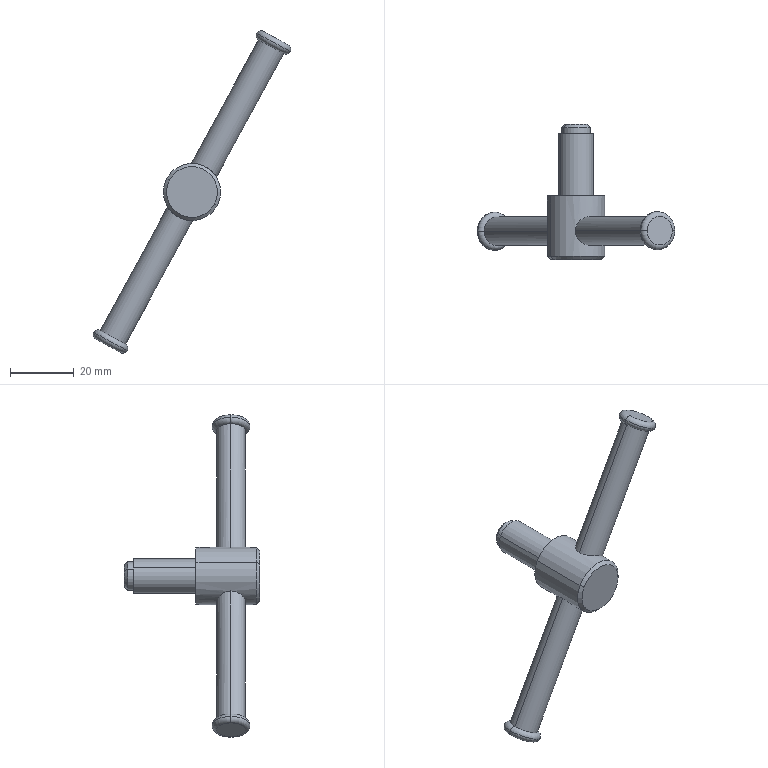Component | SolidWorks | 4-1 | 1 solid | 28 faces | box 62.09 x 42.5 x 101.27 mm | volume 13144 mm3 | cylinder 10 | torus 8 | plane 6 | cone 4 | commonest cylinder face diameters 9 x6 18 x2 10.8 x2
STEP:
#1=CARTESIAN_POINT('',(1.507,12.992,27.78));
#2=VERTEX_POINT('',#1);
#3=CARTESIAN_POINT('',(1.922,12.992,27.554));
#4=VERTEX_POINT('',#3);
#5=CARTESIAN_POINT('',(1.715,12.992,27.667));
#6=DIRECTION('',(-0.4783,-0.,-0.8782));
#7=DIRECTION('',(-0.8782,0.,0.4783));
#8=AXIS2_PLACEMENT_3D('',#5,#6,#7);
#9=CIRCLE('',#8,0.2362);
#10=EDGE_CURVE('',#2,#4,#9,.T.);
#11=ORIENTED_EDGE('',*,*,#10,.T.);
#12=CARTESIAN_POINT('',(1.842,12.992,27.53));
#13=VERTEX_POINT('',#12);
#14=CARTESIAN_POINT('',(1.87,12.992,27.582));
#15=DIRECTION('',(-0.,1.,-0.));
#16=DIRECTION('',(0.,0.,1.));
#17=AXIS2_PLACEMENT_3D('',#14,#15,#16);
#18=CIRCLE('',#17,0.05906);
#19=EDGE_CURVE('',#4,#13,#18,.T.);
#20=ORIENTED_EDGE('',*,*,#19,.T.);
#21=CARTESIAN_POINT('',(1.531,12.992,27.7));
#22=VERTEX_POINT('',#21);
#23=CARTESIAN_POINT('',(1.686,12.992,27.615));
#24=DIRECTION('',(0.4783,0.,0.8782));
#25=DIRECTION('',(0.8782,0.,-0.4783));
#26=AXIS2_PLACEMENT_3D('',#23,#24,#25);
#27=CIRCLE('',#26,0.1772);
#28=EDGE_CURVE('',#13,#22,#27,.T.);
#29=ORIENTED_EDGE('',*,*,#28,.T.);
#30=CARTESIAN_POINT('',(1.559,12.992,27.751));
#31=DIRECTION('',(0.,-1.,0.));
#32=DIRECTION('',(0.,0.,-1.));
#33=AXIS2_PLACEMENT_3D('',#30,#31,#32);
#34=CIRCLE('',#33,0.05906);
#35=EDGE_CURVE('',#2,#22,#34,.T.);
#36=ORIENTED_EDGE('',*,*,#35,.F.);
#37=EDGE_LOOP('',(#11,#20,#29,#36));
#38=FACE_OUTER_BOUND('',#37,.T.);
#39=CARTESIAN_POINT('',(1.715,12.992,27.667));
#40=DIRECTION('',(-0.4783,-0.,-0.8782));
#41=DIRECTION('',(-0.8782,-0.,0.4783));
#42=AXIS2_PLACEMENT_3D('',#39,#40,#41);
#43=TOROIDAL_SURFACE('',#42,0.1772,0.05906);
#44=ADVANCED_FACE('',(#38),#43,.T.);
#45=CARTESIAN_POINT('',(1.898,12.992,27.634));
#46=VERTEX_POINT('',#45);
#47=CARTESIAN_POINT('',(1.587,12.992,27.803));
#48=VERTEX_POINT('',#47);
#49=CARTESIAN_POINT('',(1.743,12.992,27.719));
#50=DIRECTION('',(0.4783,0.,0.8782));
#51=DIRECTION('',(-0.8782,0.,0.4783));
#52=AXIS2_PLACEMENT_3D('',#49,#50,#51);
#53=CIRCLE('',#52,0.1772);
#54=EDGE_CURVE('',#46,#48,#53,.T.);
#55=ORIENTED_EDGE('',*,*,#54,.F.);
#56=CARTESIAN_POINT('',(1.87,12.992,27.582));
#57=DIRECTION('',(-0.,1.,-0.));
#58=DIRECTION('',(0.,0.,1.));
#59=AXIS2_PLACEMENT_3D('',#56,#57,#58);
#60=CIRCLE('',#59,0.05906);
#61=EDGE_CURVE('',#46,#4,#60,.T.);
#62=ORIENTED_EDGE('',*,*,#61,.T.);
#63=ORIENTED_EDGE('',*,*,#10,.F.);
#64=CARTESIAN_POINT('',(1.559,12.992,27.751));
#65=DIRECTION('',(0.,-1.,0.));
#66=DIRECTION('',(0.,0.,-1.));
#67=AXIS2_PLACEMENT_3D('',#64,#65,#66);
#68=CIRCLE('',#67,0.05906);
#69=EDGE_CURVE('',#48,#2,#68,.T.);
#70=ORIENTED_EDGE('',*,*,#69,.F.);
#71=EDGE_LOOP('',(#55,#62,#63,#70));
#72=FACE_OUTER_BOUND('',#71,.T.);
#73=CARTESIAN_POINT('',(1.715,12.992,27.667));
#74=DIRECTION('',(-0.4783,-0.,-0.8782));
#75=DIRECTION('',(-0.8782,-0.,0.4783));
#76=AXIS2_PLACEMENT_3D('',#73,#74,#75);
#77=TOROIDAL_SURFACE('',#76,0.1772,0.05906);
#78=ADVANCED_FACE('',(#72),#77,.T.);
#79=CARTESIAN_POINT('',(1.009,12.992,26.002));
#80=VERTEX_POINT('',#79);
#81=CARTESIAN_POINT('',(0.6982,12.992,26.171));
#82=VERTEX_POINT('',#81);
#83=CARTESIAN_POINT('',(1.009,12.992,26.002));
#84=CARTESIAN_POINT('',(1.009,13.004,26.002));
#85=CARTESIAN_POINT('',(1.009,13.015,26.003));
#86=CARTESIAN_POINT('',(1.006,13.038,26.007));
#87=CARTESIAN_POINT('',(1.004,13.05,26.011));
#88=CARTESIAN_POINT('',(0.998,13.071,26.019));
#89=CARTESIAN_POINT('',(0.9946,13.081,26.024));
#90=CARTESIAN_POINT('',(0.9861,13.1,26.035));
#91=CARTESIAN_POINT('',(0.9812,13.109,26.042));
#92=CARTESIAN_POINT('',(0.97,13.125,26.055));
#93=CARTESIAN_POINT('',(0.9636,13.132,26.061));
#94=CARTESIAN_POINT('',(0.9495,13.145,26.075));
#95=CARTESIAN_POINT('',(0.9418,13.151,26.082));
#96=CARTESIAN_POINT('',(0.9251,13.16,26.096));
#97=CARTESIAN_POINT('',(0.916,13.163,26.103));
#98=CARTESIAN_POINT('',(0.8969,13.168,26.116));
#99=CARTESIAN_POINT('',(0.8869,13.169,26.122));
#100=CARTESIAN_POINT('',(0.8714,13.169,26.131));
#101=CARTESIAN_POINT('',(0.8661,13.169,26.134));
#102=CARTESIAN_POINT('',(0.8554,13.167,26.139));
#103=CARTESIAN_POINT('',(0.8501,13.167,26.141));
#104=CARTESIAN_POINT('',(0.8342,13.163,26.148));
#105=CARTESIAN_POINT('',(0.8235,13.16,26.152));
#106=CARTESIAN_POINT('',(0.8026,13.151,26.158));
#107=CARTESIAN_POINT('',(0.7925,13.145,26.161));
#108=CARTESIAN_POINT('',(0.7731,13.132,26.165));
#109=CARTESIAN_POINT('',(0.7638,13.125,26.167));
#110=CARTESIAN_POINT('',(0.7468,13.109,26.169));
#111=CARTESIAN_POINT('',(0.739,13.1,26.17));
#112=CARTESIAN_POINT('',(0.7249,13.081,26.171));
#113=CARTESIAN_POINT('',(0.7188,13.071,26.171));
#114=CARTESIAN_POINT('',(0.7088,13.05,26.171));
#115=CARTESIAN_POINT('',(0.7049,13.038,26.171));
#116=CARTESIAN_POINT('',(0.6995,13.015,26.171));
#117=CARTESIAN_POINT('',(0.6982,13.004,26.171));
#118=CARTESIAN_POINT('',(0.6982,12.992,26.171));
#119=B_SPLINE_CURVE_WITH_KNOTS('',3,(#83,#84,#85,#86,#87,#88,#89,#90,#91,#92,#93,#94,#95,#96,#97,#98,#99,#100,#101,#102,#103,#104,#105,#106,#107,#108,#109,#110,#111,#112,#113,#114,#115,#116,#117,#118),.UNSPECIFIED.,.F.,.F.,(4,2,2,2,2,2,2,2,2,2,2,2,2,2,2,2,2,4),(0.,0.0008945,0.001789,0.002684,0.003578,0.004473,0.005367,0.006262,0.007156,0.007604,0.008051,0.008945,0.00984,0.01073,0.01163,0.01252,0.01342,0.01431),.UNSPECIFIED.);
#120=EDGE_CURVE('',#80,#82,#119,.T.);
#121=ORIENTED_EDGE('',*,*,#120,.T.);
#122=CARTESIAN_POINT('',(0.5514,12.992,25.902));
#123=DIRECTION('',(0.4783,0.,0.8782));
#124=VECTOR('',#123,39.37);
#125=LINE('',#122,#124);
#126=EDGE_CURVE('',#82,#22,#125,.T.);
#127=ORIENTED_EDGE('',*,*,#126,.T.);
#128=ORIENTED_EDGE('',*,*,#28,.F.);
#129=CARTESIAN_POINT('',(0.8626,12.992,25.732));
#130=DIRECTION('',(0.4783,0.,0.8782));
#131=VECTOR('',#130,39.37);
#132=LINE('',#129,#131);
#133=EDGE_CURVE('',#80,#13,#132,.T.);
#134=ORIENTED_EDGE('',*,*,#133,.F.);
#135=EDGE_LOOP('',(#121,#127,#128,#134));
#136=FACE_OUTER_BOUND('',#135,.T.);
#137=CARTESIAN_POINT('',(0.707,12.992,25.817));
#138=DIRECTION('',(0.4783,0.,0.8782));
#139=DIRECTION('',(0.8782,0.,-0.4783));
#140=AXIS2_PLACEMENT_3D('',#137,#138,#139);
#141=CYLINDRICAL_SURFACE('',#140,0.1772);
#142=ADVANCED_FACE('',(#136),#141,.T.);
#143=CARTESIAN_POINT('',(-0.4844,12.992,24.));
#144=VERTEX_POINT('',#143);
#145=CARTESIAN_POINT('',(-0.1732,12.992,23.831));
#146=VERTEX_POINT('',#145);
#147=CARTESIAN_POINT('',(-0.3288,12.992,23.915));
#148=DIRECTION('',(-0.4783,-0.,-0.8782));
#149=DIRECTION('',(0.8782,0.,-0.4783));
#150=AXIS2_PLACEMENT_3D('',#147,#148,#149);
#151=CIRCLE('',#150,0.1772);
#152=EDGE_CURVE('',#144,#146,#151,.T.);
#153=ORIENTED_EDGE('',*,*,#152,.F.);
#154=CARTESIAN_POINT('',(-0.508,12.992,24.08));
#155=VERTEX_POINT('',#154);
#156=CARTESIAN_POINT('',(-0.4561,12.992,24.052));
#157=DIRECTION('',(0.,1.,-0.));
#158=DIRECTION('',(0.,0.,1.));
#159=AXIS2_PLACEMENT_3D('',#156,#157,#158);
#160=CIRCLE('',#159,0.05906);
#161=EDGE_CURVE('',#144,#155,#160,.T.);
#162=ORIENTED_EDGE('',*,*,#161,.T.);
#163=CARTESIAN_POINT('',(-0.09311,12.992,23.854));
#164=VERTEX_POINT('',#163);
#165=CARTESIAN_POINT('',(-0.3006,12.992,23.967));
#166=DIRECTION('',(-0.4783,-0.,-0.8782));
#167=DIRECTION('',(0.8782,0.,-0.4783));
#168=AXIS2_PLACEMENT_3D('',#165,#166,#167);
#169=CIRCLE('',#168,0.2362);
#170=EDGE_CURVE('',#155,#164,#169,.T.);
#171=ORIENTED_EDGE('',*,*,#170,.T.);
#172=CARTESIAN_POINT('',(-0.145,12.992,23.883));
#173=DIRECTION('',(0.,-1.,0.));
#174=DIRECTION('',(0.,0.,-1.));
#175=AXIS2_PLACEMENT_3D('',#172,#173,#174);
#176=CIRCLE('',#175,0.05906);
#177=EDGE_CURVE('',#146,#164,#176,.T.);
#178=ORIENTED_EDGE('',*,*,#177,.F.);
#179=EDGE_LOOP('',(#153,#162,#171,#178));
#180=FACE_OUTER_BOUND('',#179,.T.);
#181=CARTESIAN_POINT('',(-0.3006,12.992,23.967));
#182=DIRECTION('',(0.4783,0.,0.8782));
#183=DIRECTION('',(0.8782,0.,-0.4783));
#184=AXIS2_PLACEMENT_3D('',#181,#182,#183);
#185=TOROIDAL_SURFACE('',#184,0.1772,0.05906);
#186=ADVANCED_FACE('',(#180),#185,.T.);
#187=ORIENTED_EDGE('',*,*,#170,.F.);
#188=CARTESIAN_POINT('',(-0.4279,12.992,24.104));
#189=VERTEX_POINT('',#188);
#190=CARTESIAN_POINT('',(-0.4561,12.992,24.052));
#191=DIRECTION('',(0.,1.,-0.));
#192=DIRECTION('',(0.,0.,1.));
#193=AXIS2_PLACEMENT_3D('',#190,#191,#192);
#194=CIRCLE('',#193,0.05906);
#195=EDGE_CURVE('',#155,#189,#194,.T.);
#196=ORIENTED_EDGE('',*,*,#195,.T.);
#197=CARTESIAN_POINT('',(-0.1167,12.992,23.934));
#198=VERTEX_POINT('',#197);
#199=CARTESIAN_POINT('',(-0.2723,12.992,24.019));
#200=DIRECTION('',(0.4783,0.,0.8782));
#201=DIRECTION('',(0.8782,0.,-0.4783));
#202=AXIS2_PLACEMENT_3D('',#199,#200,#201);
#203=CIRCLE('',#202,0.1772);
#204=EDGE_CURVE('',#198,#189,#203,.T.);
#205=ORIENTED_EDGE('',*,*,#204,.F.);
#206=CARTESIAN_POINT('',(-0.145,12.992,23.883));
#207=DIRECTION('',(0.,-1.,0.));
#208=DIRECTION('',(0.,0.,-1.));
#209=AXIS2_PLACEMENT_3D('',#206,#207,#208);
#210=CIRCLE('',#209,0.05906);
#211=EDGE_CURVE('',#164,#198,#210,.T.);
#212=ORIENTED_EDGE('',*,*,#211,.F.);
#213=EDGE_LOOP('',(#187,#196,#205,#212));
#214=FACE_OUTER_BOUND('',#213,.T.);
#215=CARTESIAN_POINT('',(-0.3006,12.992,23.967));
#216=DIRECTION('',(0.4783,0.,0.8782));
#217=DIRECTION('',(0.8782,0.,-0.4783));
#218=AXIS2_PLACEMENT_3D('',#215,#216,#217);
#219=TOROIDAL_SURFACE('',#218,0.1772,0.05906);
#220=ADVANCED_FACE('',(#214),#219,.T.);
#221=CARTESIAN_POINT('',(0.586,14.311,25.883));
#222=VERTEX_POINT('',#221);
#223=CARTESIAN_POINT('',(0.828,14.311,25.751));
#224=VERTEX_POINT('',#223);
#225=CARTESIAN_POINT('',(0.707,14.311,25.817));
#226=DIRECTION('',(-0.,1.,-0.));
#227=DIRECTION('',(0.8782,0.,-0.4783));
#228=AXIS2_PLACEMENT_3D('',#225,#226,#227);
#229=CIRCLE('',#228,0.1378);
#230=EDGE_CURVE('',#222,#224,#229,.T.);
#231=ORIENTED_EDGE('',*,*,#230,.F.);
#232=CARTESIAN_POINT('',(0.5514,14.271,25.902));
#233=VERTEX_POINT('',#232);
#234=CARTESIAN_POINT('',(0.586,14.311,25.883));
#235=DIRECTION('',(-0.621,-0.7071,0.3382));
#236=VECTOR('',#235,39.37);
#237=LINE('',#234,#236);
#238=EDGE_CURVE('',#222,#233,#237,.T.);
#239=ORIENTED_EDGE('',*,*,#238,.T.);
#240=CARTESIAN_POINT('',(0.8626,14.271,25.732));
#241=VERTEX_POINT('',#240);
#242=CARTESIAN_POINT('',(0.707,14.271,25.817));
#243=DIRECTION('',(0.,-1.,0.));
#244=DIRECTION('',(0.8782,0.,-0.4783));
#245=AXIS2_PLACEMENT_3D('',#242,#243,#244);
#246=CIRCLE('',#245,0.1772);
#247=EDGE_CURVE('',#241,#233,#246,.T.);
#248=ORIENTED_EDGE('',*,*,#247,.F.);
#249=CARTESIAN_POINT('',(0.828,14.311,25.751));
#250=DIRECTION('',(0.621,-0.7071,-0.3382));
#251=VECTOR('',#250,39.37);
#252=LINE('',#249,#251);
#253=EDGE_CURVE('',#224,#241,#252,.T.);
#254=ORIENTED_EDGE('',*,*,#253,.F.);
#255=EDGE_LOOP('',(#231,#239,#248,#254));
#256=FACE_OUTER_BOUND('',#255,.T.);
#257=CARTESIAN_POINT('',(0.707,14.311,25.817));
#258=DIRECTION('',(0.,-1.,0.));
#259=DIRECTION('',(0.8782,0.,-0.4783));
#260=AXIS2_PLACEMENT_3D('',#257,#258,#259);
#261=CONICAL_SURFACE('',#260,0.1378,0.7854);
#262=ADVANCED_FACE('',(#256),#261,.T.);
#263=CARTESIAN_POINT('',(0.9836,12.637,25.666));
#264=VERTEX_POINT('',#263);
#265=CARTESIAN_POINT('',(0.4304,12.637,25.968));
#266=VERTEX_POINT('',#265);
#267=CARTESIAN_POINT('',(0.707,12.637,25.817));
#268=DIRECTION('',(0.,-1.,0.));
#269=DIRECTION('',(0.8782,0.,-0.4783));
#270=AXIS2_PLACEMENT_3D('',#267,#268,#269);
#271=CIRCLE('',#270,0.315);
#272=EDGE_CURVE('',#264,#266,#271,.T.);
#273=ORIENTED_EDGE('',*,*,#272,.F.);
#274=CARTESIAN_POINT('',(1.018,12.677,25.647));
#275=VERTEX_POINT('',#274);
#276=CARTESIAN_POINT('',(1.018,12.677,25.647));
#277=DIRECTION('',(0.621,0.7071,-0.3382));
#278=VECTOR('',#277,39.37);
#279=LINE('',#276,#278);
#280=EDGE_CURVE('',#264,#275,#279,.T.);
#281=ORIENTED_EDGE('',*,*,#280,.T.);
#282=CARTESIAN_POINT('',(0.3958,12.677,25.986));
#283=VERTEX_POINT('',#282);
#284=CARTESIAN_POINT('',(0.707,12.677,25.817));
#285=DIRECTION('',(-0.,1.,-0.));
#286=DIRECTION('',(0.8782,0.,-0.4783));
#287=AXIS2_PLACEMENT_3D('',#284,#285,#286);
#288=CIRCLE('',#287,0.3543);
#289=EDGE_CURVE('',#283,#275,#288,.T.);
#290=ORIENTED_EDGE('',*,*,#289,.F.);
#291=CARTESIAN_POINT('',(0.3958,12.677,25.986));
#292=DIRECTION('',(-0.621,0.7071,0.3382));
#293=VECTOR('',#292,39.37);
#294=LINE('',#291,#293);
#295=EDGE_CURVE('',#266,#283,#294,.T.);
#296=ORIENTED_EDGE('',*,*,#295,.F.);
#297=EDGE_LOOP('',(#273,#281,#290,#296));
#298=FACE_OUTER_BOUND('',#297,.T.);
#299=CARTESIAN_POINT('',(0.707,12.677,25.817));
#300=DIRECTION('',(-0.,1.,-0.));
#301=DIRECTION('',(-0.8782,0.,0.4783));
#302=AXIS2_PLACEMENT_3D('',#299,#300,#301);
#303=CONICAL_SURFACE('',#302,0.3543,0.7854);
#304=ADVANCED_FACE('',(#298),#303,.T.);
#305=CARTESIAN_POINT('',(0.5514,14.193,25.902));
#306=VERTEX_POINT('',#305);
#307=CARTESIAN_POINT('',(0.8626,14.193,25.732));
#308=VERTEX_POINT('',#307);
#309=CARTESIAN_POINT('',(0.707,14.193,25.817));
#310=DIRECTION('',(-0.,1.,-0.));
#311=DIRECTION('',(-0.8782,0.,0.4783));
#312=AXIS2_PLACEMENT_3D('',#309,#310,#311);
#313=CIRCLE('',#312,0.1772);
#314=EDGE_CURVE('',#306,#308,#313,.T.);
#315=ORIENTED_EDGE('',*,*,#314,.T.);
#316=CARTESIAN_POINT('',(0.8626,14.193,25.732));
#317=DIRECTION('',(-0.,1.,-0.));
#318=VECTOR('',#317,39.37);
#319=LINE('',#316,#318);
#320=EDGE_CURVE('',#308,#241,#319,.T.);
#321=ORIENTED_EDGE('',*,*,#320,.T.);
#322=ORIENTED_EDGE('',*,*,#247,.T.);
#323=CARTESIAN_POINT('',(0.5514,14.193,25.902));
#324=DIRECTION('',(-0.,1.,-0.));
#325=VECTOR('',#324,39.37);
#326=LINE('',#323,#325);
#327=EDGE_CURVE('',#306,#233,#326,.T.);
#328=ORIENTED_EDGE('',*,*,#327,.F.);
#329=EDGE_LOOP('',(#315,#321,#322,#328));
#330=FACE_OUTER_BOUND('',#329,.T.);
#331=CARTESIAN_POINT('',(0.707,14.193,25.817));
#332=DIRECTION('',(-0.,1.,-0.));
#333=DIRECTION('',(-0.8782,0.,0.4783));
#334=AXIS2_PLACEMENT_3D('',#331,#332,#333);
#335=CYLINDRICAL_SURFACE('',#334,0.1772);
#336=ADVANCED_FACE('',(#330),#335,.T.);
#337=ORIENTED_EDGE('',*,*,#120,.F.);
#338=CARTESIAN_POINT('',(0.6982,12.992,26.171));
#339=CARTESIAN_POINT('',(0.6982,12.98,26.171));
#340=CARTESIAN_POINT('',(0.6996,12.968,26.171));
#341=CARTESIAN_POINT('',(0.7049,12.945,26.171));
#342=CARTESIAN_POINT('',(0.7088,12.934,26.171));
#343=CARTESIAN_POINT('',(0.719,12.913,26.171));
#344=CARTESIAN_POINT('',(0.7251,12.902,26.171));
#345=CARTESIAN_POINT('',(0.739,12.883,26.17));
#346=CARTESIAN_POINT('',(0.747,12.875,26.169));
#347=CARTESIAN_POINT('',(0.764,12.858,26.167));
#348=CARTESIAN_POINT('',(0.7731,12.851,26.165));
#349=CARTESIAN_POINT('',(0.7925,12.838,26.161));
#350=CARTESIAN_POINT('',(0.8028,12.833,26.158));
#351=CARTESIAN_POINT('',(0.8234,12.824,26.152));
#352=CARTESIAN_POINT('',(0.834,12.821,26.148));
#353=CARTESIAN_POINT('',(0.8554,12.816,26.139));
#354=CARTESIAN_POINT('',(0.866,12.815,26.134));
#355=CARTESIAN_POINT('',(0.8815,12.815,26.125));
#356=CARTESIAN_POINT('',(0.8866,12.815,26.122));
#357=CARTESIAN_POINT('',(0.8966,12.816,26.116));
#358=CARTESIAN_POINT('',(0.9016,12.817,26.113));
#359=CARTESIAN_POINT('',(0.916,12.82,26.103));
#360=CARTESIAN_POINT('',(0.9249,12.824,26.097));
#361=CARTESIAN_POINT('',(0.9418,12.833,26.083));
#362=CARTESIAN_POINT('',(0.9496,12.838,26.075));
#363=CARTESIAN_POINT('',(0.9636,12.851,26.061));
#364=CARTESIAN_POINT('',(0.97,12.859,26.055));
#365=CARTESIAN_POINT('',(0.9812,12.875,26.041));
#366=CARTESIAN_POINT('',(0.9861,12.883,26.035));
#367=CARTESIAN_POINT('',(0.9945,12.902,26.024));
#368=CARTESIAN_POINT('',(0.9981,12.913,26.019));
#369=CARTESIAN_POINT('',(1.004,12.934,26.011));
#370=CARTESIAN_POINT('',(1.006,12.945,26.007));
#371=CARTESIAN_POINT('',(1.009,12.968,26.003));
#372=CARTESIAN_POINT('',(1.009,12.98,26.002));
#373=CARTESIAN_POINT('',(1.009,12.992,26.002));
#374=B_SPLINE_CURVE_WITH_KNOTS('',3,(#338,#339,#340,#341,#342,#343,#344,#345,#346,#347,#348,#349,#350,#351,#352,#353,#354,#355,#356,#357,#358,#359,#360,#361,#362,#363,#364,#365,#366,#367,#368,#369,#370,#371,#372,#373),.UNSPECIFIED.,.F.,.F.,(4,2,2,2,2,2,2,2,2,2,2,2,2,2,2,2,2,4),(0.01431,0.01521,0.0161,0.01699,0.01788,0.01878,0.01967,0.02056,0.02146,0.0219,0.02235,0.02324,0.02414,0.02503,0.02592,0.02681,0.02771,0.0286),.UNSPECIFIED.);
#375=EDGE_CURVE('',#82,#80,#374,.T.);
#376=ORIENTED_EDGE('',*,*,#375,.F.);
#377=EDGE_LOOP('',(#337,#376));
#378=FACE_BOUND('',#377,.T.);
#379=ORIENTED_EDGE('',*,*,#289,.T.);
#380=CARTESIAN_POINT('',(1.018,13.425,25.647));
#381=VERTEX_POINT('',#380);
#382=CARTESIAN_POINT('',(1.018,12.637,25.647));
#383=DIRECTION('',(-0.,1.,-0.));
#384=VECTOR('',#383,39.37);
#385=LINE('',#382,#384);
#386=EDGE_CURVE('',#275,#381,#385,.T.);
#387=ORIENTED_EDGE('',*,*,#386,.T.);
#388=CARTESIAN_POINT('',(0.3958,13.425,25.986));
#389=VERTEX_POINT('',#388);
#390=CARTESIAN_POINT('',(0.707,13.425,25.817));
#391=DIRECTION('',(-0.,1.,-0.));
#392=DIRECTION('',(-0.8782,0.,0.4783));
#393=AXIS2_PLACEMENT_3D('',#390,#391,#392);
#394=CIRCLE('',#393,0.3543);
#395=EDGE_CURVE('',#389,#381,#394,.T.);
#396=ORIENTED_EDGE('',*,*,#395,.F.);
#397=CARTESIAN_POINT('',(0.3958,12.637,25.986));
#398=DIRECTION('',(-0.,1.,-0.));
#399=VECTOR('',#398,39.37);
#400=LINE('',#397,#399);
#401=EDGE_CURVE('',#283,#389,#400,.T.);
#402=ORIENTED_EDGE('',*,*,#401,.F.);
#403=EDGE_LOOP('',(#379,#387,#396,#402));
#404=FACE_OUTER_BOUND('',#403,.T.);
#405=CARTESIAN_POINT('',(0.707,12.637,25.817));
#406=DIRECTION('',(-0.,1.,-0.));
#407=DIRECTION('',(-0.8782,0.,0.4783));
#408=AXIS2_PLACEMENT_3D('',#405,#406,#407);
#409=CYLINDRICAL_SURFACE('',#408,0.3543);
#410=ADVANCED_FACE('',(#378,#404),#409,.T.);
#411=CARTESIAN_POINT('',(0.4046,12.992,25.632));
#412=VERTEX_POINT('',#411);
#413=CARTESIAN_POINT('',(0.7158,12.992,25.463));
#414=VERTEX_POINT('',#413);
#415=CARTESIAN_POINT('',(0.4046,12.992,25.632));
#416=CARTESIAN_POINT('',(0.4046,13.004,25.632));
#417=CARTESIAN_POINT('',(0.4053,13.015,25.631));
#418=CARTESIAN_POINT('',(0.4081,13.038,25.627));
#419=CARTESIAN_POINT('',(0.4103,13.05,25.623));
#420=CARTESIAN_POINT('',(0.4159,13.071,25.615));
#421=CARTESIAN_POINT('',(0.4194,13.081,25.61));
#422=CARTESIAN_POINT('',(0.4279,13.1,25.599));
#423=CARTESIAN_POINT('',(0.4328,13.109,25.592));
#424=CARTESIAN_POINT('',(0.444,13.125,25.579));
#425=CARTESIAN_POINT('',(0.4503,13.132,25.572));
#426=CARTESIAN_POINT('',(0.4645,13.145,25.558));
#427=CARTESIAN_POINT('',(0.4721,13.151,25.551));
#428=CARTESIAN_POINT('',(0.4888,13.16,25.538));
#429=CARTESIAN_POINT('',(0.498,13.163,25.531));
#430=CARTESIAN_POINT('',(0.5171,13.168,25.518));
#431=CARTESIAN_POINT('',(0.527,13.169,25.511));
#432=CARTESIAN_POINT('',(0.5426,13.169,25.503));
#433=CARTESIAN_POINT('',(0.5479,13.169,25.5));
#434=CARTESIAN_POINT('',(0.5585,13.167,25.495));
#435=CARTESIAN_POINT('',(0.5638,13.167,25.493));
#436=CARTESIAN_POINT('',(0.5798,13.163,25.486));
#437=CARTESIAN_POINT('',(0.5905,13.16,25.482));
#438=CARTESIAN_POINT('',(0.6114,13.151,25.476));
#439=CARTESIAN_POINT('',(0.6215,13.145,25.473));
#440=CARTESIAN_POINT('',(0.6409,13.132,25.469));
#441=CARTESIAN_POINT('',(0.6502,13.125,25.467));
#442=CARTESIAN_POINT('',(0.6672,13.109,25.465));
#443=CARTESIAN_POINT('',(0.675,13.1,25.464));
#444=CARTESIAN_POINT('',(0.6891,13.081,25.463));
#445=CARTESIAN_POINT('',(0.6951,13.071,25.463));
#446=CARTESIAN_POINT('',(0.7051,13.05,25.463));
#447=CARTESIAN_POINT('',(0.7091,13.038,25.463));
#448=CARTESIAN_POINT('',(0.7144,13.015,25.463));
#449=CARTESIAN_POINT('',(0.7158,13.004,25.463));
#450=CARTESIAN_POINT('',(0.7158,12.992,25.463));
#451=B_SPLINE_CURVE_WITH_KNOTS('',3,(#415,#416,#417,#418,#419,#420,#421,#422,#423,#424,#425,#426,#427,#428,#429,#430,#431,#432,#433,#434,#435,#436,#437,#438,#439,#440,#441,#442,#443,#444,#445,#446,#447,#448,#449,#450),.UNSPECIFIED.,.F.,.F.,(4,2,2,2,2,2,2,2,2,2,2,2,2,2,2,2,2,4),(0.,0.0008945,0.001789,0.002684,0.003578,0.004473,0.005367,0.006262,0.007156,0.007604,0.008051,0.008945,0.00984,0.01073,0.01163,0.01252,0.01342,0.01431),.UNSPECIFIED.);
#452=EDGE_CURVE('',#412,#414,#451,.T.);
#453=ORIENTED_EDGE('',*,*,#452,.T.);
#454=CARTESIAN_POINT('',(0.8626,12.992,25.732));
#455=DIRECTION('',(-0.4783,-0.,-0.8782));
#456=VECTOR('',#455,39.37);
#457=LINE('',#454,#456);
#458=EDGE_CURVE('',#414,#198,#457,.T.);
#459=ORIENTED_EDGE('',*,*,#458,.T.);
#460=ORIENTED_EDGE('',*,*,#204,.T.);
#461=CARTESIAN_POINT('',(0.5514,12.992,25.902));
#462=DIRECTION('',(-0.4783,-0.,-0.8782));
#463=VECTOR('',#462,39.37);
#464=LINE('',#461,#463);
#465=EDGE_CURVE('',#412,#189,#464,.T.);
#466=ORIENTED_EDGE('',*,*,#465,.F.);
#467=EDGE_LOOP('',(#453,#459,#460,#466));
#468=FACE_OUTER_BOUND('',#467,.T.);
#469=CARTESIAN_POINT('',(0.707,12.992,25.817));
#470=DIRECTION('',(-0.4783,-0.,-0.8782));
#471=DIRECTION('',(-0.8782,0.,0.4783));
#472=AXIS2_PLACEMENT_3D('',#469,#470,#471);
#473=CYLINDRICAL_SURFACE('',#472,0.1772);
#474=ADVANCED_FACE('',(#468),#473,.T.);
#475=CARTESIAN_POINT('',(0.8937,14.193,25.715));
#476=VERTEX_POINT('',#475);
#477=CARTESIAN_POINT('',(0.5203,14.193,25.919));
#478=VERTEX_POINT('',#477);
#479=CARTESIAN_POINT('',(0.707,14.193,25.817));
#480=DIRECTION('',(0.,-1.,0.));
#481=DIRECTION('',(-0.8782,0.,0.4783));
#482=AXIS2_PLACEMENT_3D('',#479,#480,#481);
#483=CIRCLE('',#482,0.2126);
#484=EDGE_CURVE('',#476,#478,#483,.T.);
#485=ORIENTED_EDGE('',*,*,#484,.T.);
#486=CARTESIAN_POINT('',(0.5203,13.425,25.919));
#487=VERTEX_POINT('',#486);
#488=CARTESIAN_POINT('',(0.5203,14.311,25.919));
#489=DIRECTION('',(0.,-1.,0.));
#490=VECTOR('',#489,39.37);
#491=LINE('',#488,#490);
#492=EDGE_CURVE('',#478,#487,#491,.T.);
#493=ORIENTED_EDGE('',*,*,#492,.T.);
#494=CARTESIAN_POINT('',(0.8937,13.425,25.715));
#495=VERTEX_POINT('',#494);
#496=CARTESIAN_POINT('',(0.707,13.425,25.817));
#497=DIRECTION('',(0.,-1.,0.));
#498=DIRECTION('',(-0.8782,0.,0.4783));
#499=AXIS2_PLACEMENT_3D('',#496,#497,#498);
#500=CIRCLE('',#499,0.2126);
#501=EDGE_CURVE('',#495,#487,#500,.T.);
#502=ORIENTED_EDGE('',*,*,#501,.F.);
#503=CARTESIAN_POINT('',(0.8937,14.311,25.715));
#504=DIRECTION('',(0.,-1.,0.));
#505=VECTOR('',#504,39.37);
#506=LINE('',#503,#505);
#507=EDGE_CURVE('',#476,#495,#506,.T.);
#508=ORIENTED_EDGE('',*,*,#507,.F.);
#509=EDGE_LOOP('',(#485,#493,#502,#508));
#510=FACE_OUTER_BOUND('',#509,.T.);
#511=CARTESIAN_POINT('',(0.707,14.311,25.817));
#512=DIRECTION('',(0.,-1.,0.));
#513=DIRECTION('',(0.8782,0.,-0.4783));
#514=AXIS2_PLACEMENT_3D('',#511,#512,#513);
#515=CYLINDRICAL_SURFACE('',#514,0.2126);
#516=ADVANCED_FACE('',(#510),#515,.T.);
#517=ORIENTED_EDGE('',*,*,#492,.F.);
#518=CARTESIAN_POINT('',(0.707,14.193,25.817));
#519=DIRECTION('',(0.,-1.,0.));
#520=DIRECTION('',(-0.8782,0.,0.4783));
#521=AXIS2_PLACEMENT_3D('',#518,#519,#520);
#522=CIRCLE('',#521,0.2126);
#523=EDGE_CURVE('',#478,#476,#522,.T.);
#524=ORIENTED_EDGE('',*,*,#523,.T.);
#525=ORIENTED_EDGE('',*,*,#507,.T.);
#526=CARTESIAN_POINT('',(0.707,13.425,25.817));
#527=DIRECTION('',(0.,-1.,0.));
#528=DIRECTION('',(-0.8782,0.,0.4783));
#529=AXIS2_PLACEMENT_3D('',#526,#527,#528);
#530=CIRCLE('',#529,0.2126);
#531=EDGE_CURVE('',#487,#495,#530,.T.);
#532=ORIENTED_EDGE('',*,*,#531,.F.);
#533=EDGE_LOOP('',(#517,#524,#525,#532));
#534=FACE_OUTER_BOUND('',#533,.T.);
#535=CARTESIAN_POINT('',(0.707,14.311,25.817));
#536=DIRECTION('',(0.,-1.,0.));
#537=DIRECTION('',(0.8782,0.,-0.4783));
#538=AXIS2_PLACEMENT_3D('',#535,#536,#537);
#539=CYLINDRICAL_SURFACE('',#538,0.2126);
#540=ADVANCED_FACE('',(#534),#539,.T.);
#541=CARTESIAN_POINT('',(-0.3288,12.992,23.915));
#542=DIRECTION('',(-0.4783,-0.,-0.8782));
#543=DIRECTION('',(0.8782,0.,-0.4783));
#544=AXIS2_PLACEMENT_3D('',#541,#542,#543);
#545=CIRCLE('',#544,0.1772);
#546=EDGE_CURVE('',#146,#144,#545,.T.);
#547=ORIENTED_EDGE('',*,*,#546,.T.);
#548=ORIENTED_EDGE('',*,*,#152,.T.);
#549=EDGE_LOOP('',(#547,#548));
#550=FACE_OUTER_BOUND('',#549,.T.);
#551=CARTESIAN_POINT('',(-0.3288,12.992,23.915));
#552=DIRECTION('',(0.4783,0.,0.8782));
#553=DIRECTION('',(0.8782,-0.,-0.4783));
#554=AXIS2_PLACEMENT_3D('',#551,#552,#553);
#555=PLANE('',#554);
#556=ADVANCED_FACE('',(#550),#555,.F.);
#557=ORIENTED_EDGE('',*,*,#458,.F.);
#558=CARTESIAN_POINT('',(0.7158,12.992,25.463));
#559=CARTESIAN_POINT('',(0.7158,12.98,25.463));
#560=CARTESIAN_POINT('',(0.7144,12.968,25.463));
#561=CARTESIAN_POINT('',(0.7091,12.945,25.463));
#562=CARTESIAN_POINT('',(0.7052,12.934,25.463));
#563=CARTESIAN_POINT('',(0.695,12.913,25.463));
#564=CARTESIAN_POINT('',(0.6889,12.902,25.463));
#565=CARTESIAN_POINT('',(0.6749,12.883,25.464));
#566=CARTESIAN_POINT('',(0.667,12.875,25.465));
#567=CARTESIAN_POINT('',(0.6499,12.858,25.467));
#568=CARTESIAN_POINT('',(0.6408,12.851,25.469));
#569=CARTESIAN_POINT('',(0.6215,12.838,25.473));
#570=CARTESIAN_POINT('',(0.6112,12.833,25.476));
#571=CARTESIAN_POINT('',(0.5905,12.824,25.482));
#572=CARTESIAN_POINT('',(0.58,12.821,25.486));
#573=CARTESIAN_POINT('',(0.5586,12.816,25.495));
#574=CARTESIAN_POINT('',(0.5479,12.815,25.5));
#575=CARTESIAN_POINT('',(0.5325,12.815,25.509));
#576=CARTESIAN_POINT('',(0.5274,12.815,25.511));
#577=CARTESIAN_POINT('',(0.5173,12.816,25.518));
#578=CARTESIAN_POINT('',(0.5124,12.817,25.521));
#579=CARTESIAN_POINT('',(0.498,12.82,25.531));
#580=CARTESIAN_POINT('',(0.489,12.824,25.537));
#581=CARTESIAN_POINT('',(0.4722,12.833,25.551));
#582=CARTESIAN_POINT('',(0.4644,12.838,25.559));
#583=CARTESIAN_POINT('',(0.4504,12.851,25.572));
#584=CARTESIAN_POINT('',(0.444,12.859,25.579));
#585=CARTESIAN_POINT('',(0.4327,12.875,25.592));
#586=CARTESIAN_POINT('',(0.4279,12.883,25.599));
#587=CARTESIAN_POINT('',(0.4195,12.902,25.61));
#588=CARTESIAN_POINT('',(0.4159,12.913,25.615));
#589=CARTESIAN_POINT('',(0.4103,12.934,25.623));
#590=CARTESIAN_POINT('',(0.4082,12.945,25.626));
#591=CARTESIAN_POINT('',(0.4053,12.968,25.631));
#592=CARTESIAN_POINT('',(0.4046,12.98,25.632));
#593=CARTESIAN_POINT('',(0.4046,12.992,25.632));
#594=B_SPLINE_CURVE_WITH_KNOTS('',3,(#558,#559,#560,#561,#562,#563,#564,#565,#566,#567,#568,#569,#570,#571,#572,#573,#574,#575,#576,#577,#578,#579,#580,#581,#582,#583,#584,#585,#586,#587,#588,#589,#590,#591,#592,#593),.UNSPECIFIED.,.F.,.F.,(4,2,2,2,2,2,2,2,2,2,2,2,2,2,2,2,2,4),(0.01431,0.01521,0.0161,0.01699,0.01788,0.01878,0.01967,0.02056,0.02146,0.0219,0.02235,0.02324,0.02414,0.02503,0.02592,0.02681,0.02771,0.0286),.UNSPECIFIED.);
#595=EDGE_CURVE('',#414,#412,#594,.T.);
#596=ORIENTED_EDGE('',*,*,#595,.T.);
#597=ORIENTED_EDGE('',*,*,#465,.T.);
#598=CARTESIAN_POINT('',(-0.2723,12.992,24.019));
#599=DIRECTION('',(0.4783,0.,0.8782));
#600=DIRECTION('',(0.8782,0.,-0.4783));
#601=AXIS2_PLACEMENT_3D('',#598,#599,#600);
#602=CIRCLE('',#601,0.1772);
#603=EDGE_CURVE('',#189,#198,#602,.T.);
#604=ORIENTED_EDGE('',*,*,#603,.T.);
#605=EDGE_LOOP('',(#557,#596,#597,#604));
#606=FACE_OUTER_BOUND('',#605,.T.);
#607=CARTESIAN_POINT('',(0.707,12.992,25.817));
#608=DIRECTION('',(-0.4783,-0.,-0.8782));
#609=DIRECTION('',(-0.8782,0.,0.4783));
#610=AXIS2_PLACEMENT_3D('',#607,#608,#609);
#611=CYLINDRICAL_SURFACE('',#610,0.1772);
#612=ADVANCED_FACE('',(#606),#611,.T.);
#613=ORIENTED_EDGE('',*,*,#386,.F.);
#614=CARTESIAN_POINT('',(0.707,12.677,25.817));
#615=DIRECTION('',(-0.,1.,-0.));
#616=DIRECTION('',(0.8782,0.,-0.4783));
#617=AXIS2_PLACEMENT_3D('',#614,#615,#616);
#618=CIRCLE('',#617,0.3543);
#619=EDGE_CURVE('',#275,#283,#618,.T.);
#620=ORIENTED_EDGE('',*,*,#619,.T.);
#621=ORIENTED_EDGE('',*,*,#401,.T.);
#622=CARTESIAN_POINT('',(0.707,13.425,25.817));
#623=DIRECTION('',(-0.,1.,-0.));
#624=DIRECTION('',(-0.8782,0.,0.4783));
#625=AXIS2_PLACEMENT_3D('',#622,#623,#624);
#626=CIRCLE('',#625,0.3543);
#627=EDGE_CURVE('',#381,#389,#626,.T.);
#628=ORIENTED_EDGE('',*,*,#627,.F.);
#629=EDGE_LOOP('',(#613,#620,#621,#628));
#630=FACE_OUTER_BOUND('',#629,.T.);
#631=ORIENTED_EDGE('',*,*,#452,.F.);
#632=ORIENTED_EDGE('',*,*,#595,.F.);
#633=EDGE_LOOP('',(#631,#632));
#634=FACE_BOUND('',#633,.T.);
#635=CARTESIAN_POINT('',(0.707,12.637,25.817));
#636=DIRECTION('',(-0.,1.,-0.));
#637=DIRECTION('',(-0.8782,0.,0.4783));
#638=AXIS2_PLACEMENT_3D('',#635,#636,#637);
#639=CYLINDRICAL_SURFACE('',#638,0.3543);
#640=ADVANCED_FACE('',(#630,#634),#639,.T.);
#641=ORIENTED_EDGE('',*,*,#501,.T.);
#642=ORIENTED_EDGE('',*,*,#531,.T.);
#643=EDGE_LOOP('',(#641,#642));
#644=FACE_BOUND('',#643,.T.);
#645=ORIENTED_EDGE('',*,*,#395,.T.);
#646=ORIENTED_EDGE('',*,*,#627,.T.);
#647=EDGE_LOOP('',(#645,#646));
#648=FACE_OUTER_BOUND('',#647,.T.);
#649=CARTESIAN_POINT('',(0.707,13.425,25.817));
#650=DIRECTION('',(-0.,1.,-0.));
#651=DIRECTION('',(-0.8782,0.,0.4783));
#652=AXIS2_PLACEMENT_3D('',#649,#650,#651);
#653=PLANE('',#652);
#654=ADVANCED_FACE('',(#644,#648),#653,.T.);
#655=CARTESIAN_POINT('',(0.707,12.637,25.817));
#656=DIRECTION('',(0.,-1.,0.));
#657=DIRECTION('',(0.8782,0.,-0.4783));
#658=AXIS2_PLACEMENT_3D('',#655,#656,#657);
#659=CIRCLE('',#658,0.315);
#660=EDGE_CURVE('',#266,#264,#659,.T.);
#661=ORIENTED_EDGE('',*,*,#660,.T.);
#662=ORIENTED_EDGE('',*,*,#272,.T.);
#663=EDGE_LOOP('',(#661,#662));
#664=FACE_OUTER_BOUND('',#663,.T.);
#665=CARTESIAN_POINT('',(0.707,12.637,25.817));
#666=DIRECTION('',(0.,-1.,0.));
#667=DIRECTION('',(0.8782,-0.,-0.4783));
#668=AXIS2_PLACEMENT_3D('',#665,#666,#667);
#669=PLANE('',#668);
#670=ADVANCED_FACE('',(#664),#669,.T.);
#671=ORIENTED_EDGE('',*,*,#484,.F.);
#672=ORIENTED_EDGE('',*,*,#523,.F.);
#673=EDGE_LOOP('',(#671,#672));
#674=FACE_OUTER_BOUND('',#673,.T.);
#675=ORIENTED_EDGE('',*,*,#314,.F.);
#676=CARTESIAN_POINT('',(0.707,14.193,25.817));
#677=DIRECTION('',(-0.,1.,-0.));
#678=DIRECTION('',(-0.8782,0.,0.4783));
#679=AXIS2_PLACEMENT_3D('',#676,#677,#678);
#680=CIRCLE('',#679,0.1772);
#681=EDGE_CURVE('',#308,#306,#680,.T.);
#682=ORIENTED_EDGE('',*,*,#681,.F.);
#683=EDGE_LOOP('',(#675,#682));
#684=FACE_BOUND('',#683,.T.);
#685=CARTESIAN_POINT('',(0.2738,14.193,25.022));
#686=DIRECTION('',(-0.,1.,-0.));
#687=DIRECTION('',(-0.8782,0.,0.4783));
#688=AXIS2_PLACEMENT_3D('',#685,#686,#687);
#689=PLANE('',#688);
#690=ADVANCED_FACE('',(#674,#684),#689,.T.);
#691=ORIENTED_EDGE('',*,*,#320,.F.);
#692=ORIENTED_EDGE('',*,*,#681,.T.);
#693=ORIENTED_EDGE('',*,*,#327,.T.);
#694=CARTESIAN_POINT('',(0.707,14.271,25.817));
#695=DIRECTION('',(0.,-1.,0.));
#696=DIRECTION('',(0.8782,0.,-0.4783));
#697=AXIS2_PLACEMENT_3D('',#694,#695,#696);
#698=CIRCLE('',#697,0.1772);
#699=EDGE_CURVE('',#233,#241,#698,.T.);
#700=ORIENTED_EDGE('',*,*,#699,.T.);
#701=EDGE_LOOP('',(#691,#692,#693,#700));
#702=FACE_OUTER_BOUND('',#701,.T.);
#703=CARTESIAN_POINT('',(0.707,14.193,25.817));
#704=DIRECTION('',(-0.,1.,-0.));
#705=DIRECTION('',(-0.8782,0.,0.4783));
#706=AXIS2_PLACEMENT_3D('',#703,#704,#705);
#707=CYLINDRICAL_SURFACE('',#706,0.1772);
#708=ADVANCED_FACE('',(#702),#707,.T.);
#709=CARTESIAN_POINT('',(0.707,14.311,25.817));
#710=DIRECTION('',(-0.,1.,-0.));
#711=DIRECTION('',(0.8782,0.,-0.4783));
#712=AXIS2_PLACEMENT_3D('',#709,#710,#711);
#713=CIRCLE('',#712,0.1378);
#714=EDGE_CURVE('',#224,#222,#713,.T.);
#715=ORIENTED_EDGE('',*,*,#714,.T.);
#716=ORIENTED_EDGE('',*,*,#230,.T.);
#717=EDGE_LOOP('',(#715,#716));
#718=FACE_OUTER_BOUND('',#717,.T.);
#719=CARTESIAN_POINT('',(0.707,14.311,25.817));
#720=DIRECTION('',(0.,-1.,0.));
#721=DIRECTION('',(0.8782,-0.,-0.4783));
#722=AXIS2_PLACEMENT_3D('',#719,#720,#721);
#723=PLANE('',#722);
#724=ADVANCED_FACE('',(#718),#723,.F.);
#725=ORIENTED_EDGE('',*,*,#280,.F.);
#726=ORIENTED_EDGE('',*,*,#660,.F.);
#727=ORIENTED_EDGE('',*,*,#295,.T.);
#728=ORIENTED_EDGE('',*,*,#619,.F.);
#729=EDGE_LOOP('',(#725,#726,#727,#728));
#730=FACE_OUTER_BOUND('',#729,.T.);
#731=CARTESIAN_POINT('',(0.707,12.677,25.817));
#732=DIRECTION('',(-0.,1.,-0.));
#733=DIRECTION('',(-0.8782,0.,0.4783));
#734=AXIS2_PLACEMENT_3D('',#731,#732,#733);
#735=CONICAL_SURFACE('',#734,0.3543,0.7854);
#736=ADVANCED_FACE('',(#730),#735,.T.);
#737=ORIENTED_EDGE('',*,*,#238,.F.);
#738=ORIENTED_EDGE('',*,*,#714,.F.);
#739=ORIENTED_EDGE('',*,*,#253,.T.);
#740=ORIENTED_EDGE('',*,*,#699,.F.);
#741=EDGE_LOOP('',(#737,#738,#739,#740));
#742=FACE_OUTER_BOUND('',#741,.T.);
#743=CARTESIAN_POINT('',(0.707,14.311,25.817));
#744=DIRECTION('',(0.,-1.,0.));
#745=DIRECTION('',(0.8782,0.,-0.4783));
#746=AXIS2_PLACEMENT_3D('',#743,#744,#745);
#747=CONICAL_SURFACE('',#746,0.1378,0.7854);
#748=ADVANCED_FACE('',(#742),#747,.T.);
#749=ORIENTED_EDGE('',*,*,#195,.F.);
#750=CARTESIAN_POINT('',(-0.3006,12.992,23.967));
#751=DIRECTION('',(-0.4783,-0.,-0.8782));
#752=DIRECTION('',(0.8782,0.,-0.4783));
#753=AXIS2_PLACEMENT_3D('',#750,#751,#752);
#754=CIRCLE('',#753,0.2362);
#755=EDGE_CURVE('',#164,#155,#754,.T.);
#756=ORIENTED_EDGE('',*,*,#755,.F.);
#757=ORIENTED_EDGE('',*,*,#211,.T.);
#758=ORIENTED_EDGE('',*,*,#603,.F.);
#759=EDGE_LOOP('',(#749,#756,#757,#758));
#760=FACE_OUTER_BOUND('',#759,.T.);
#761=CARTESIAN_POINT('',(-0.3006,12.992,23.967));
#762=DIRECTION('',(0.4783,0.,0.8782));
#763=DIRECTION('',(0.8782,0.,-0.4783));
#764=AXIS2_PLACEMENT_3D('',#761,#762,#763);
#765=TOROIDAL_SURFACE('',#764,0.1772,0.05906);
#766=ADVANCED_FACE('',(#760),#765,.T.);
#767=ORIENTED_EDGE('',*,*,#161,.F.);
#768=ORIENTED_EDGE('',*,*,#546,.F.);
#769=ORIENTED_EDGE('',*,*,#177,.T.);
#770=ORIENTED_EDGE('',*,*,#755,.T.);
#771=EDGE_LOOP('',(#767,#768,#769,#770));
#772=FACE_OUTER_BOUND('',#771,.T.);
#773=CARTESIAN_POINT('',(-0.3006,12.992,23.967));
#774=DIRECTION('',(0.4783,0.,0.8782));
#775=DIRECTION('',(0.8782,0.,-0.4783));
#776=AXIS2_PLACEMENT_3D('',#773,#774,#775);
#777=TOROIDAL_SURFACE('',#776,0.1772,0.05906);
#778=ADVANCED_FACE('',(#772),#777,.T.);
#779=ORIENTED_EDGE('',*,*,#126,.F.);
#780=ORIENTED_EDGE('',*,*,#375,.T.);
#781=ORIENTED_EDGE('',*,*,#133,.T.);
#782=CARTESIAN_POINT('',(1.686,12.992,27.615));
#783=DIRECTION('',(0.4783,0.,0.8782));
#784=DIRECTION('',(0.8782,0.,-0.4783));
#785=AXIS2_PLACEMENT_3D('',#782,#783,#784);
#786=CIRCLE('',#785,0.1772);
#787=EDGE_CURVE('',#22,#13,#786,.T.);
#788=ORIENTED_EDGE('',*,*,#787,.F.);
#789=EDGE_LOOP('',(#779,#780,#781,#788));
#790=FACE_OUTER_BOUND('',#789,.T.);
#791=CARTESIAN_POINT('',(0.707,12.992,25.817));
#792=DIRECTION('',(0.4783,0.,0.8782));
#793=DIRECTION('',(0.8782,0.,-0.4783));
#794=AXIS2_PLACEMENT_3D('',#791,#792,#793);
#795=CYLINDRICAL_SURFACE('',#794,0.1772);
#796=ADVANCED_FACE('',(#790),#795,.T.);
#797=CARTESIAN_POINT('',(1.743,12.992,27.719));
#798=DIRECTION('',(0.4783,0.,0.8782));
#799=DIRECTION('',(-0.8782,0.,0.4783));
#800=AXIS2_PLACEMENT_3D('',#797,#798,#799);
#801=CIRCLE('',#800,0.1772);
#802=EDGE_CURVE('',#48,#46,#801,.T.);
#803=ORIENTED_EDGE('',*,*,#802,.T.);
#804=ORIENTED_EDGE('',*,*,#54,.T.);
#805=EDGE_LOOP('',(#803,#804));
#806=FACE_OUTER_BOUND('',#805,.T.);
#807=CARTESIAN_POINT('',(1.743,12.992,27.719));
#808=DIRECTION('',(-0.4783,-0.,-0.8782));
#809=DIRECTION('',(0.8782,-0.,-0.4783));
#810=AXIS2_PLACEMENT_3D('',#807,#808,#809);
#811=PLANE('',#810);
#812=ADVANCED_FACE('',(#806),#811,.F.);
#813=ORIENTED_EDGE('',*,*,#61,.F.);
#814=ORIENTED_EDGE('',*,*,#802,.F.);
#815=ORIENTED_EDGE('',*,*,#69,.T.);
#816=CARTESIAN_POINT('',(1.715,12.992,27.667));
#817=DIRECTION('',(-0.4783,-0.,-0.8782));
#818=DIRECTION('',(-0.8782,0.,0.4783));
#819=AXIS2_PLACEMENT_3D('',#816,#817,#818);
#820=CIRCLE('',#819,0.2362);
#821=EDGE_CURVE('',#4,#2,#820,.T.);
#822=ORIENTED_EDGE('',*,*,#821,.F.);
#823=EDGE_LOOP('',(#813,#814,#815,#822));
#824=FACE_OUTER_BOUND('',#823,.T.);
#825=CARTESIAN_POINT('',(1.715,12.992,27.667));
#826=DIRECTION('',(-0.4783,-0.,-0.8782));
#827=DIRECTION('',(-0.8782,-0.,0.4783));
#828=AXIS2_PLACEMENT_3D('',#825,#826,#827);
#829=TOROIDAL_SURFACE('',#828,0.1772,0.05906);
#830=ADVANCED_FACE('',(#824),#829,.T.);
#831=ORIENTED_EDGE('',*,*,#19,.F.);
#832=ORIENTED_EDGE('',*,*,#821,.T.);
#833=ORIENTED_EDGE('',*,*,#35,.T.);
#834=ORIENTED_EDGE('',*,*,#787,.T.);
#835=EDGE_LOOP('',(#831,#832,#833,#834));
#836=FACE_OUTER_BOUND('',#835,.T.);
#837=CARTESIAN_POINT('',(1.715,12.992,27.667));
#838=DIRECTION('',(-0.4783,-0.,-0.8782));
#839=DIRECTION('',(-0.8782,-0.,0.4783));
#840=AXIS2_PLACEMENT_3D('',#837,#838,#839);
#841=TOROIDAL_SURFACE('',#840,0.1772,0.05906);
#842=ADVANCED_FACE('',(#836),#841,.T.);
#843=CLOSED_SHELL('',(#44,#78,#142,#186,#220,#262,#304,#336,#410,#474,#516,#540,#556,#612,#640,#654,#670,#690,#708,#724,#736,#748,#766,#778,#796,#812,#830,#842));
#844=MANIFOLD_SOLID_BREP('',#843);
#845=CARTESIAN_POINT('',(0.,0.,0.));
#846=DIRECTION('',(0.,0.,1.));
#847=DIRECTION('',(1.,0.,0.));
#848=AXIS2_PLACEMENT_3D('',#845,#846,#847);
#849=(LENGTH_UNIT()NAMED_UNIT(*)SI_UNIT($,.METRE.));
#850=LENGTH_MEASURE_WITH_UNIT(LENGTH_MEASURE(0.0254),#849);
#851=DIMENSIONAL_EXPONENTS(1.,0.,0.,0.,0.,0.,0.);
#852=(CONVERSION_BASED_UNIT('',#850)LENGTH_UNIT()NAMED_UNIT(#851));
#853=UNCERTAINTY_MEASURE_WITH_UNIT(LENGTH_MEASURE(0.00001),#852,'','');
#854=(NAMED_UNIT(*)PLANE_ANGLE_UNIT()SI_UNIT($,.RADIAN.));
#855=(NAMED_UNIT(*)SI_UNIT($,.STERADIAN.)SOLID_ANGLE_UNIT());
#856=(GEOMETRIC_REPRESENTATION_CONTEXT(3)GLOBAL_UNCERTAINTY_ASSIGNED_CONTEXT((#853))GLOBAL_UNIT_ASSIGNED_CONTEXT((#852,#854,#855))REPRESENTATION_CONTEXT('',''));
#857=ADVANCED_BREP_SHAPE_REPRESENTATION('',(#844,#848),#856);
#858=COLOUR_RGB('',0.7922,0.8196,0.9333);
#859=FILL_AREA_STYLE_COLOUR('',#858);
#860=FILL_AREA_STYLE('',(#859));
#861=SURFACE_STYLE_FILL_AREA(#860);
#862=SURFACE_SIDE_STYLE('',(#861));
#863=SURFACE_STYLE_USAGE(.BOTH.,#862);
#864=PRESENTATION_STYLE_ASSIGNMENT((#863));
#865=STYLED_ITEM('',(#864),#844);
#866=(LENGTH_UNIT()NAMED_UNIT(*)SI_UNIT($,.METRE.));
#867=LENGTH_MEASURE_WITH_UNIT(LENGTH_MEASURE(0.0254),#866);
#868=DIMENSIONAL_EXPONENTS(1.,0.,0.,0.,0.,0.,0.);
#869=(CONVERSION_BASED_UNIT('',#867)LENGTH_UNIT()NAMED_UNIT(#868));
#870=UNCERTAINTY_MEASURE_WITH_UNIT(LENGTH_MEASURE(0.00001),#869,'','');
#871=(NAMED_UNIT(*)PLANE_ANGLE_UNIT()SI_UNIT($,.RADIAN.));
#872=(NAMED_UNIT(*)SI_UNIT($,.STERADIAN.)SOLID_ANGLE_UNIT());
#873=(GEOMETRIC_REPRESENTATION_CONTEXT(3)GLOBAL_UNCERTAINTY_ASSIGNED_CONTEXT((#870))GLOBAL_UNIT_ASSIGNED_CONTEXT((#869,#871,#872))REPRESENTATION_CONTEXT('',''));
#874=MECHANICAL_DESIGN_GEOMETRIC_PRESENTATION_REPRESENTATION('',(#865),#873);
#875=PRESENTATION_LAYER_ASSIGNMENT('','',(#865));